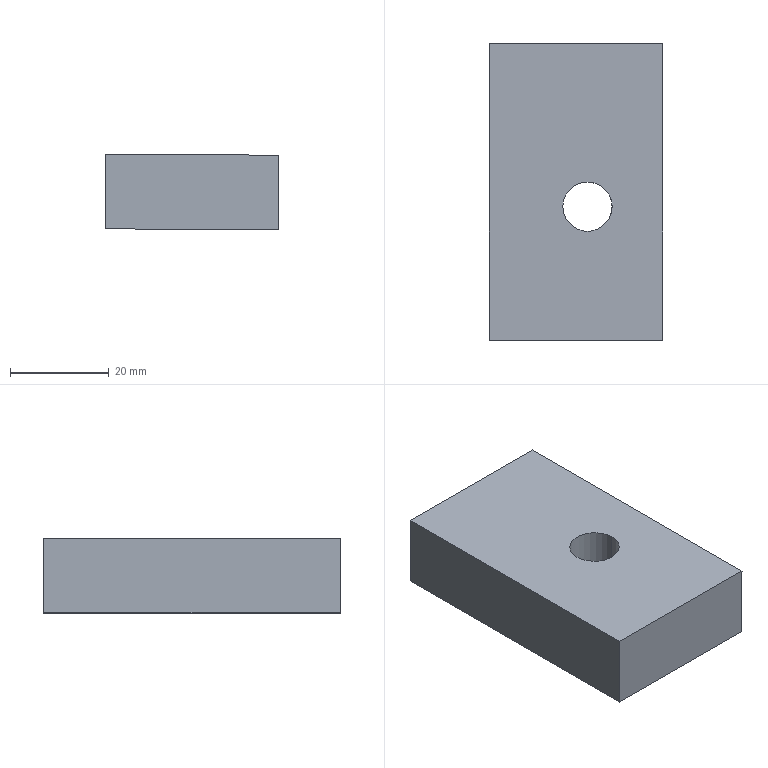Component | SolidWorks | TelescopicCylinderConnectionBlock-1 | 1 solid | 8 faces | box 35.02 x 60 x 15.04 mm | volume 30322 mm3 | plane 6 | cylinder 2 | commonest cylinder face diameters 10 x2
build123d program:
from build123d import *

# Parameters (mm, degrees)
SKETCH1_W           = 35
SKETCH1_H           = 15
BOSS_EXTRUDE1_DEPTH = 60
M10_TAPPED_HOLE1_D  = 10


with BuildPart() as part:
    # Sketch1 → Boss-Extrude1 (new body)
    with BuildSketch(Plane(origin=(0, 0, 0), x_dir=(1, 0, 0), z_dir=(0, 1, 0))):
        Rectangle(SKETCH1_W, SKETCH1_H)
    extrude(amount=BOSS_EXTRUDE1_DEPTH)

    # M10 Tapped Hole1 (through all)
    with Locations(Plane.XY.offset(7.5)):
        with Locations((2.32, 27.042)):
            Hole(M10_TAPPED_HOLE1_D / 2)


solid = part.part

# Placed as in the assembly
solid = solid.moved(Location((-98.088, 844.54, 1067.223), (0, 0.0619, 0)))
STEP:
#1=CARTESIAN_POINT('',(-3.968,34.314,41.722));
#2=VERTEX_POINT('',#1);
#3=CARTESIAN_POINT('',(-3.574,34.314,41.721));
#4=VERTEX_POINT('',#3);
#5=CARTESIAN_POINT('',(-3.771,34.314,41.721));
#6=DIRECTION('',(0.00108,0.,1.));
#7=DIRECTION('',(1.,0.,-0.00108));
#8=AXIS2_PLACEMENT_3D('',#5,#6,#7);
#9=CIRCLE('',#8,0.1969);
#10=EDGE_CURVE('',#2,#4,#9,.T.);
#11=ORIENTED_EDGE('',*,*,#10,.F.);
#12=CARTESIAN_POINT('',(-3.967,34.314,42.312));
#13=VERTEX_POINT('',#12);
#14=CARTESIAN_POINT('',(-3.967,34.314,42.312));
#15=DIRECTION('',(0.00108,0.,1.));
#16=VECTOR('',#15,39.37);
#17=LINE('',#14,#16);
#18=EDGE_CURVE('',#2,#13,#17,.T.);
#19=ORIENTED_EDGE('',*,*,#18,.T.);
#20=CARTESIAN_POINT('',(-3.573,34.314,42.312));
#21=VERTEX_POINT('',#20);
#22=CARTESIAN_POINT('',(-3.77,34.314,42.312));
#23=DIRECTION('',(0.00108,0.,1.));
#24=DIRECTION('',(1.,0.,-0.00108));
#25=AXIS2_PLACEMENT_3D('',#22,#23,#24);
#26=CIRCLE('',#25,0.1969);
#27=EDGE_CURVE('',#13,#21,#26,.T.);
#28=ORIENTED_EDGE('',*,*,#27,.T.);
#29=CARTESIAN_POINT('',(-3.573,34.314,42.312));
#30=DIRECTION('',(0.00108,0.,1.));
#31=VECTOR('',#30,39.37);
#32=LINE('',#29,#31);
#33=EDGE_CURVE('',#4,#21,#32,.T.);
#34=ORIENTED_EDGE('',*,*,#33,.F.);
#35=EDGE_LOOP('',(#11,#19,#28,#34));
#36=FACE_OUTER_BOUND('',#35,.T.);
#37=CARTESIAN_POINT('',(-3.77,34.314,42.312));
#38=DIRECTION('',(0.00108,0.,1.));
#39=DIRECTION('',(1.,0.,-0.00108));
#40=AXIS2_PLACEMENT_3D('',#37,#38,#39);
#41=CYLINDRICAL_SURFACE('',#40,0.1969);
#42=ADVANCED_FACE('',(#36),#41,.F.);
#43=CARTESIAN_POINT('',(-3.172,33.25,42.311));
#44=VERTEX_POINT('',#43);
#45=CARTESIAN_POINT('',(-3.173,33.25,41.721));
#46=VERTEX_POINT('',#45);
#47=CARTESIAN_POINT('',(-3.172,33.25,42.311));
#48=DIRECTION('',(-0.00108,-0.,-1.));
#49=VECTOR('',#48,39.37);
#50=LINE('',#47,#49);
#51=EDGE_CURVE('',#44,#46,#50,.T.);
#52=ORIENTED_EDGE('',*,*,#51,.T.);
#53=CARTESIAN_POINT('',(-3.173,35.612,41.721));
#54=VERTEX_POINT('',#53);
#55=CARTESIAN_POINT('',(-3.173,35.612,41.721));
#56=DIRECTION('',(0.,-1.,0.));
#57=VECTOR('',#56,39.37);
#58=LINE('',#55,#57);
#59=EDGE_CURVE('',#54,#46,#58,.T.);
#60=ORIENTED_EDGE('',*,*,#59,.F.);
#61=CARTESIAN_POINT('',(-3.172,35.612,42.311));
#62=VERTEX_POINT('',#61);
#63=CARTESIAN_POINT('',(-3.172,35.612,42.311));
#64=DIRECTION('',(-0.00108,-0.,-1.));
#65=VECTOR('',#64,39.37);
#66=LINE('',#63,#65);
#67=EDGE_CURVE('',#62,#54,#66,.T.);
#68=ORIENTED_EDGE('',*,*,#67,.F.);
#69=CARTESIAN_POINT('',(-3.172,35.612,42.311));
#70=DIRECTION('',(0.,-1.,0.));
#71=VECTOR('',#70,39.37);
#72=LINE('',#69,#71);
#73=EDGE_CURVE('',#62,#44,#72,.T.);
#74=ORIENTED_EDGE('',*,*,#73,.T.);
#75=EDGE_LOOP('',(#52,#60,#68,#74));
#76=FACE_OUTER_BOUND('',#75,.T.);
#77=CARTESIAN_POINT('',(-3.172,35.612,42.311));
#78=DIRECTION('',(-1.,-0.,0.00108));
#79=DIRECTION('',(0.00108,0.,1.));
#80=AXIS2_PLACEMENT_3D('',#77,#78,#79);
#81=PLANE('',#80);
#82=ADVANCED_FACE('',(#76),#81,.F.);
#83=CARTESIAN_POINT('',(-3.771,34.314,41.721));
#84=DIRECTION('',(0.00108,0.,1.));
#85=DIRECTION('',(1.,0.,-0.00108));
#86=AXIS2_PLACEMENT_3D('',#83,#84,#85);
#87=CIRCLE('',#86,0.1969);
#88=EDGE_CURVE('',#4,#2,#87,.T.);
#89=ORIENTED_EDGE('',*,*,#88,.T.);
#90=ORIENTED_EDGE('',*,*,#10,.T.);
#91=EDGE_LOOP('',(#89,#90));
#92=FACE_BOUND('',#91,.T.);
#93=CARTESIAN_POINT('',(-4.551,33.25,41.722));
#94=VERTEX_POINT('',#93);
#95=CARTESIAN_POINT('',(-4.551,33.25,41.722));
#96=DIRECTION('',(-1.,-0.,0.00108));
#97=VECTOR('',#96,39.37);
#98=LINE('',#95,#97);
#99=EDGE_CURVE('',#46,#94,#98,.T.);
#100=ORIENTED_EDGE('',*,*,#99,.T.);
#101=CARTESIAN_POINT('',(-4.551,35.612,41.722));
#102=VERTEX_POINT('',#101);
#103=CARTESIAN_POINT('',(-4.551,35.612,41.722));
#104=DIRECTION('',(0.,-1.,0.));
#105=VECTOR('',#104,39.37);
#106=LINE('',#103,#105);
#107=EDGE_CURVE('',#102,#94,#106,.T.);
#108=ORIENTED_EDGE('',*,*,#107,.F.);
#109=CARTESIAN_POINT('',(-4.551,35.612,41.722));
#110=DIRECTION('',(-1.,-0.,0.00108));
#111=VECTOR('',#110,39.37);
#112=LINE('',#109,#111);
#113=EDGE_CURVE('',#54,#102,#112,.T.);
#114=ORIENTED_EDGE('',*,*,#113,.F.);
#115=ORIENTED_EDGE('',*,*,#59,.T.);
#116=EDGE_LOOP('',(#100,#108,#114,#115));
#117=FACE_OUTER_BOUND('',#116,.T.);
#118=CARTESIAN_POINT('',(-4.551,35.612,41.722));
#119=DIRECTION('',(0.00108,0.,1.));
#120=DIRECTION('',(1.,0.,-0.00108));
#121=AXIS2_PLACEMENT_3D('',#118,#119,#120);
#122=PLANE('',#121);
#123=ADVANCED_FACE('',(#92,#117),#122,.F.);
#124=CARTESIAN_POINT('',(-4.55,33.25,42.313));
#125=VERTEX_POINT('',#124);
#126=CARTESIAN_POINT('',(-4.55,33.25,42.313));
#127=DIRECTION('',(0.00108,0.,1.));
#128=VECTOR('',#127,39.37);
#129=LINE('',#126,#128);
#130=EDGE_CURVE('',#94,#125,#129,.T.);
#131=ORIENTED_EDGE('',*,*,#130,.T.);
#132=CARTESIAN_POINT('',(-4.55,35.612,42.313));
#133=VERTEX_POINT('',#132);
#134=CARTESIAN_POINT('',(-4.55,35.612,42.313));
#135=DIRECTION('',(0.,-1.,0.));
#136=VECTOR('',#135,39.37);
#137=LINE('',#134,#136);
#138=EDGE_CURVE('',#133,#125,#137,.T.);
#139=ORIENTED_EDGE('',*,*,#138,.F.);
#140=CARTESIAN_POINT('',(-4.55,35.612,42.313));
#141=DIRECTION('',(0.00108,0.,1.));
#142=VECTOR('',#141,39.37);
#143=LINE('',#140,#142);
#144=EDGE_CURVE('',#102,#133,#143,.T.);
#145=ORIENTED_EDGE('',*,*,#144,.F.);
#146=ORIENTED_EDGE('',*,*,#107,.T.);
#147=EDGE_LOOP('',(#131,#139,#145,#146));
#148=FACE_OUTER_BOUND('',#147,.T.);
#149=CARTESIAN_POINT('',(-4.55,35.612,42.313));
#150=DIRECTION('',(1.,0.,-0.00108));
#151=DIRECTION('',(-0.00108,-0.,-1.));
#152=AXIS2_PLACEMENT_3D('',#149,#150,#151);
#153=PLANE('',#152);
#154=ADVANCED_FACE('',(#148),#153,.F.);
#155=CARTESIAN_POINT('',(-3.77,34.314,42.312));
#156=DIRECTION('',(0.00108,0.,1.));
#157=DIRECTION('',(1.,0.,-0.00108));
#158=AXIS2_PLACEMENT_3D('',#155,#156,#157);
#159=CIRCLE('',#158,0.1969);
#160=EDGE_CURVE('',#21,#13,#159,.T.);
#161=ORIENTED_EDGE('',*,*,#160,.F.);
#162=ORIENTED_EDGE('',*,*,#27,.F.);
#163=EDGE_LOOP('',(#161,#162));
#164=FACE_BOUND('',#163,.T.);
#165=CARTESIAN_POINT('',(-4.55,33.25,42.313));
#166=DIRECTION('',(1.,0.,-0.00108));
#167=VECTOR('',#166,39.37);
#168=LINE('',#165,#167);
#169=EDGE_CURVE('',#125,#44,#168,.T.);
#170=ORIENTED_EDGE('',*,*,#169,.T.);
#171=ORIENTED_EDGE('',*,*,#73,.F.);
#172=CARTESIAN_POINT('',(-4.55,35.612,42.313));
#173=DIRECTION('',(1.,0.,-0.00108));
#174=VECTOR('',#173,39.37);
#175=LINE('',#172,#174);
#176=EDGE_CURVE('',#133,#62,#175,.T.);
#177=ORIENTED_EDGE('',*,*,#176,.F.);
#178=ORIENTED_EDGE('',*,*,#138,.T.);
#179=EDGE_LOOP('',(#170,#171,#177,#178));
#180=FACE_OUTER_BOUND('',#179,.T.);
#181=CARTESIAN_POINT('',(-4.55,35.612,42.313));
#182=DIRECTION('',(-0.00108,-0.,-1.));
#183=DIRECTION('',(-1.,-0.,0.00108));
#184=AXIS2_PLACEMENT_3D('',#181,#182,#183);
#185=PLANE('',#184);
#186=ADVANCED_FACE('',(#164,#180),#185,.F.);
#187=ORIENTED_EDGE('',*,*,#67,.T.);
#188=ORIENTED_EDGE('',*,*,#113,.T.);
#189=ORIENTED_EDGE('',*,*,#144,.T.);
#190=ORIENTED_EDGE('',*,*,#176,.T.);
#191=EDGE_LOOP('',(#187,#188,#189,#190));
#192=FACE_OUTER_BOUND('',#191,.T.);
#193=CARTESIAN_POINT('',(-3.862,35.612,42.017));
#194=DIRECTION('',(0.,-1.,0.));
#195=DIRECTION('',(-0.00108,-0.,-1.));
#196=AXIS2_PLACEMENT_3D('',#193,#194,#195);
#197=PLANE('',#196);
#198=ADVANCED_FACE('',(#192),#197,.F.);
#199=ORIENTED_EDGE('',*,*,#51,.F.);
#200=ORIENTED_EDGE('',*,*,#169,.F.);
#201=ORIENTED_EDGE('',*,*,#130,.F.);
#202=ORIENTED_EDGE('',*,*,#99,.F.);
#203=EDGE_LOOP('',(#199,#200,#201,#202));
#204=FACE_OUTER_BOUND('',#203,.T.);
#205=CARTESIAN_POINT('',(-3.862,33.25,42.017));
#206=DIRECTION('',(0.,-1.,0.));
#207=DIRECTION('',(-0.00108,-0.,-1.));
#208=AXIS2_PLACEMENT_3D('',#205,#206,#207);
#209=PLANE('',#208);
#210=ADVANCED_FACE('',(#204),#209,.T.);
#211=ORIENTED_EDGE('',*,*,#18,.F.);
#212=ORIENTED_EDGE('',*,*,#88,.F.);
#213=ORIENTED_EDGE('',*,*,#33,.T.);
#214=ORIENTED_EDGE('',*,*,#160,.T.);
#215=EDGE_LOOP('',(#211,#212,#213,#214));
#216=FACE_OUTER_BOUND('',#215,.T.);
#217=CARTESIAN_POINT('',(-3.77,34.314,42.312));
#218=DIRECTION('',(0.00108,0.,1.));
#219=DIRECTION('',(1.,0.,-0.00108));
#220=AXIS2_PLACEMENT_3D('',#217,#218,#219);
#221=CYLINDRICAL_SURFACE('',#220,0.1969);
#222=ADVANCED_FACE('',(#216),#221,.F.);
#223=CLOSED_SHELL('',(#42,#82,#123,#154,#186,#198,#210,#222));
#224=MANIFOLD_SOLID_BREP('',#223);
#225=CARTESIAN_POINT('',(0.,0.,0.));
#226=DIRECTION('',(0.,0.,1.));
#227=DIRECTION('',(1.,0.,0.));
#228=AXIS2_PLACEMENT_3D('',#225,#226,#227);
#229=(LENGTH_UNIT()NAMED_UNIT(*)SI_UNIT($,.METRE.));
#230=LENGTH_MEASURE_WITH_UNIT(LENGTH_MEASURE(0.0254),#229);
#231=DIMENSIONAL_EXPONENTS(1.,0.,0.,0.,0.,0.,0.);
#232=(CONVERSION_BASED_UNIT('',#230)LENGTH_UNIT()NAMED_UNIT(#231));
#233=UNCERTAINTY_MEASURE_WITH_UNIT(LENGTH_MEASURE(0.00001),#232,'','');
#234=(NAMED_UNIT(*)PLANE_ANGLE_UNIT()SI_UNIT($,.RADIAN.));
#235=(NAMED_UNIT(*)SI_UNIT($,.STERADIAN.)SOLID_ANGLE_UNIT());
#236=(GEOMETRIC_REPRESENTATION_CONTEXT(3)GLOBAL_UNCERTAINTY_ASSIGNED_CONTEXT((#233))GLOBAL_UNIT_ASSIGNED_CONTEXT((#232,#234,#235))REPRESENTATION_CONTEXT('',''));
#237=ADVANCED_BREP_SHAPE_REPRESENTATION('',(#224,#228),#236);
#238=COLOUR_RGB('',0.7922,0.8196,0.9333);
#239=FILL_AREA_STYLE_COLOUR('',#238);
#240=FILL_AREA_STYLE('',(#239));
#241=SURFACE_STYLE_FILL_AREA(#240);
#242=SURFACE_SIDE_STYLE('',(#241));
#243=SURFACE_STYLE_USAGE(.BOTH.,#242);
#244=PRESENTATION_STYLE_ASSIGNMENT((#243));
#245=STYLED_ITEM('',(#244),#224);
#246=(LENGTH_UNIT()NAMED_UNIT(*)SI_UNIT($,.METRE.));
#247=LENGTH_MEASURE_WITH_UNIT(LENGTH_MEASURE(0.0254),#246);
#248=DIMENSIONAL_EXPONENTS(1.,0.,0.,0.,0.,0.,0.);
#249=(CONVERSION_BASED_UNIT('',#247)LENGTH_UNIT()NAMED_UNIT(#248));
#250=UNCERTAINTY_MEASURE_WITH_UNIT(LENGTH_MEASURE(0.00001),#249,'','');
#251=(NAMED_UNIT(*)PLANE_ANGLE_UNIT()SI_UNIT($,.RADIAN.));
#252=(NAMED_UNIT(*)SI_UNIT($,.STERADIAN.)SOLID_ANGLE_UNIT());
#253=(GEOMETRIC_REPRESENTATION_CONTEXT(3)GLOBAL_UNCERTAINTY_ASSIGNED_CONTEXT((#250))GLOBAL_UNIT_ASSIGNED_CONTEXT((#249,#251,#252))REPRESENTATION_CONTEXT('',''));
#254=MECHANICAL_DESIGN_GEOMETRIC_PRESENTATION_REPRESENTATION('',(#245),#253);
#255=PRESENTATION_LAYER_ASSIGNMENT('','',(#245));